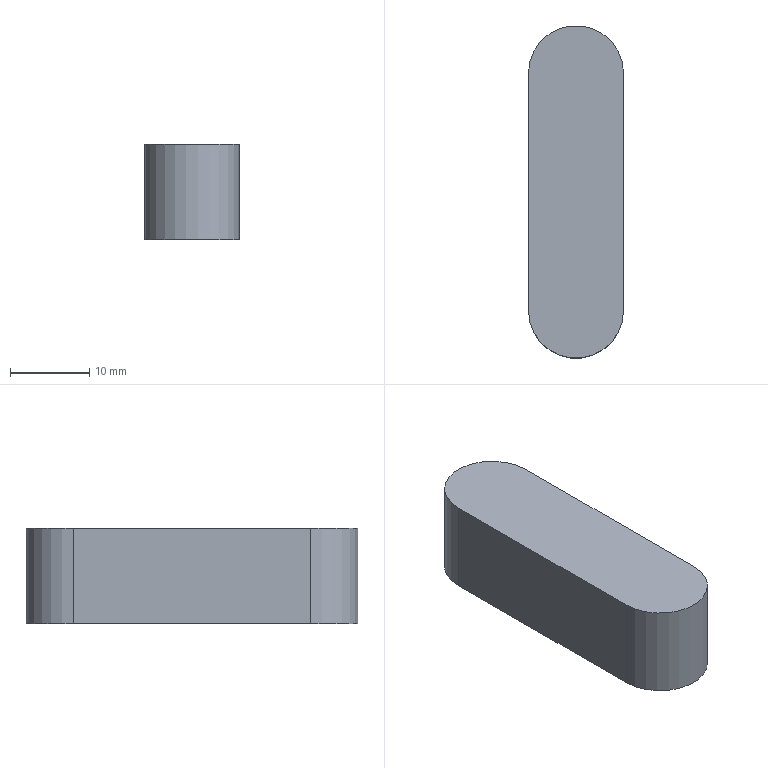Component | NX | KEY1 | 1 solid | 6 faces | box 12 x 42 x 12 mm | volume 5677 mm3 | plane 4 | cylinder 2 | commonest cylinder face diameters 12 x2
STEP:
#1=CARTESIAN_POINT('',(0.,0.,0.));
#2=DIRECTION('',(0.,0.,1.));
#3=DIRECTION('',(1.,0.,0.));
#4=AXIS2_PLACEMENT_3D('',#1,#2,#3);
#5=CARTESIAN_POINT('',(-122.42,193.257,48.472));
#6=VERTEX_POINT('',#5);
#7=CARTESIAN_POINT('',(-122.42,163.257,48.472));
#8=VERTEX_POINT('',#7);
#9=CARTESIAN_POINT('',(-122.42,178.257,48.472));
#10=DIRECTION('',(0.,-1.,0.));
#11=VECTOR('',#10,1.);
#12=LINE('',#9,#11);
#13=CARTESIAN_POINT('',(-128.42,178.257,48.472));
#14=DIRECTION('',(0.,0.,1.));
#15=DIRECTION('',(0.,-1.,0.));
#16=AXIS2_PLACEMENT_3D('',#13,#14,#15);
#17=PLANE('',#16);
#18=CARTESIAN_POINT('',(0.,6.));
#19=DIRECTION('',(1.,0.));
#20=VECTOR('',#19,1.);
#21=LINE('',#18,#20);
#22=(GEOMETRIC_REPRESENTATION_CONTEXT(2)PARAMETRIC_REPRESENTATION_CONTEXT()REPRESENTATION_CONTEXT('',''));
#23=DEFINITIONAL_REPRESENTATION('',(#21),#22);
#24=PCURVE('',#17,#23);
#25=CARTESIAN_POINT('',(-122.42,178.257,36.472));
#26=DIRECTION('',(1.,0.,0.));
#27=DIRECTION('',(0.,0.,1.));
#28=AXIS2_PLACEMENT_3D('',#25,#26,#27);
#29=PLANE('',#28);
#30=CARTESIAN_POINT('',(12.,0.));
#31=DIRECTION('',(0.,1.));
#32=VECTOR('',#31,1.);
#33=LINE('',#30,#32);
#34=(GEOMETRIC_REPRESENTATION_CONTEXT(2)PARAMETRIC_REPRESENTATION_CONTEXT()REPRESENTATION_CONTEXT('',''));
#35=DEFINITIONAL_REPRESENTATION('',(#33),#34);
#36=PCURVE('',#29,#35);
#37=SURFACE_CURVE('',#12,(#24,#36),.PCURVE_S1.);
#38=EDGE_CURVE('',#6,#8,#37,.T.);
#39=ORIENTED_EDGE('',*,*,#38,.F.);
#40=CARTESIAN_POINT('',(-134.42,193.257,48.472));
#41=VERTEX_POINT('',#40);
#42=CARTESIAN_POINT('',(-128.42,193.257,48.472));
#43=DIRECTION('',(0.,0.,1.));
#44=DIRECTION('',(0.,-1.,0.));
#45=AXIS2_PLACEMENT_3D('',#42,#43,#44);
#46=CIRCLE('',#45,6.);
#47=CARTESIAN_POINT('',(-15.,0.));
#48=DIRECTION('',(1.,0.));
#49=AXIS2_PLACEMENT_2D('',#47,#48);
#50=CIRCLE('',#49,6.);
#51=(GEOMETRIC_REPRESENTATION_CONTEXT(2)PARAMETRIC_REPRESENTATION_CONTEXT()REPRESENTATION_CONTEXT('',''));
#52=DEFINITIONAL_REPRESENTATION('',(#50),#51);
#53=PCURVE('',#17,#52);
#54=CARTESIAN_POINT('',(-128.42,193.257,36.472));
#55=DIRECTION('',(0.,0.,1.));
#56=DIRECTION('',(0.,-1.,0.));
#57=AXIS2_PLACEMENT_3D('',#54,#55,#56);
#58=CYLINDRICAL_SURFACE('',#57,6.);
#59=CARTESIAN_POINT('',(0.,12.));
#60=DIRECTION('',(1.,0.));
#61=VECTOR('',#60,1.);
#62=LINE('',#59,#61);
#63=(GEOMETRIC_REPRESENTATION_CONTEXT(2)PARAMETRIC_REPRESENTATION_CONTEXT()REPRESENTATION_CONTEXT('',''));
#64=DEFINITIONAL_REPRESENTATION('',(#62),#63);
#65=PCURVE('',#58,#64);
#66=SURFACE_CURVE('',#46,(#53,#65),.PCURVE_S1.);
#67=EDGE_CURVE('',#6,#41,#66,.T.);
#68=ORIENTED_EDGE('',*,*,#67,.T.);
#69=CARTESIAN_POINT('',(-134.42,163.257,48.472));
#70=VERTEX_POINT('',#69);
#71=CARTESIAN_POINT('',(-134.42,178.257,48.472));
#72=DIRECTION('',(0.,1.,0.));
#73=VECTOR('',#72,1.);
#74=LINE('',#71,#73);
#75=CARTESIAN_POINT('',(0.,-6.));
#76=DIRECTION('',(-1.,0.));
#77=VECTOR('',#76,1.);
#78=LINE('',#75,#77);
#79=(GEOMETRIC_REPRESENTATION_CONTEXT(2)PARAMETRIC_REPRESENTATION_CONTEXT()REPRESENTATION_CONTEXT('',''));
#80=DEFINITIONAL_REPRESENTATION('',(#78),#79);
#81=PCURVE('',#17,#80);
#82=CARTESIAN_POINT('',(-134.42,178.257,36.472));
#83=DIRECTION('',(-1.,0.,0.));
#84=DIRECTION('',(0.,0.,-1.));
#85=AXIS2_PLACEMENT_3D('',#82,#83,#84);
#86=PLANE('',#85);
#87=CARTESIAN_POINT('',(-12.,0.));
#88=DIRECTION('',(0.,-1.));
#89=VECTOR('',#88,1.);
#90=LINE('',#87,#89);
#91=(GEOMETRIC_REPRESENTATION_CONTEXT(2)PARAMETRIC_REPRESENTATION_CONTEXT()REPRESENTATION_CONTEXT('',''));
#92=DEFINITIONAL_REPRESENTATION('',(#90),#91);
#93=PCURVE('',#86,#92);
#94=SURFACE_CURVE('',#74,(#81,#93),.PCURVE_S1.);
#95=EDGE_CURVE('',#70,#41,#94,.T.);
#96=ORIENTED_EDGE('',*,*,#95,.F.);
#97=CARTESIAN_POINT('',(-128.42,163.257,48.472));
#98=DIRECTION('',(0.,0.,1.));
#99=DIRECTION('',(0.,-1.,0.));
#100=AXIS2_PLACEMENT_3D('',#97,#98,#99);
#101=CIRCLE('',#100,6.);
#102=CARTESIAN_POINT('',(15.,0.));
#103=DIRECTION('',(1.,0.));
#104=AXIS2_PLACEMENT_2D('',#102,#103);
#105=CIRCLE('',#104,6.);
#106=(GEOMETRIC_REPRESENTATION_CONTEXT(2)PARAMETRIC_REPRESENTATION_CONTEXT()REPRESENTATION_CONTEXT('',''));
#107=DEFINITIONAL_REPRESENTATION('',(#105),#106);
#108=PCURVE('',#17,#107);
#109=CARTESIAN_POINT('',(-128.42,163.257,36.472));
#110=DIRECTION('',(0.,0.,1.));
#111=DIRECTION('',(0.,-1.,0.));
#112=AXIS2_PLACEMENT_3D('',#109,#110,#111);
#113=CYLINDRICAL_SURFACE('',#112,6.);
#114=CARTESIAN_POINT('',(0.,12.));
#115=DIRECTION('',(1.,0.));
#116=VECTOR('',#115,1.);
#117=LINE('',#114,#116);
#118=(GEOMETRIC_REPRESENTATION_CONTEXT(2)PARAMETRIC_REPRESENTATION_CONTEXT()REPRESENTATION_CONTEXT('',''));
#119=DEFINITIONAL_REPRESENTATION('',(#117),#118);
#120=PCURVE('',#113,#119);
#121=SURFACE_CURVE('',#101,(#108,#120),.PCURVE_S1.);
#122=EDGE_CURVE('',#70,#8,#121,.T.);
#123=ORIENTED_EDGE('',*,*,#122,.T.);
#124=EDGE_LOOP('',(#39,#68,#96,#123));
#125=FACE_BOUND('',#124,.T.);
#126=ADVANCED_FACE('',(#125),#17,.T.);
#127=ORIENTED_EDGE('',*,*,#95,.T.);
#128=CARTESIAN_POINT('',(-134.42,193.257,36.472));
#129=VERTEX_POINT('',#128);
#130=CARTESIAN_POINT('',(-134.42,193.257,36.472));
#131=DIRECTION('',(0.,0.,-1.));
#132=VECTOR('',#131,1.);
#133=LINE('',#130,#132);
#134=CARTESIAN_POINT('',(0.,-15.));
#135=DIRECTION('',(1.,0.));
#136=VECTOR('',#135,1.);
#137=LINE('',#134,#136);
#138=(GEOMETRIC_REPRESENTATION_CONTEXT(2)PARAMETRIC_REPRESENTATION_CONTEXT()REPRESENTATION_CONTEXT('',''));
#139=DEFINITIONAL_REPRESENTATION('',(#137),#138);
#140=PCURVE('',#86,#139);
#141=CARTESIAN_POINT('',(4.712,0.));
#142=DIRECTION('',(0.,-1.));
#143=VECTOR('',#142,1.);
#144=LINE('',#141,#143);
#145=(GEOMETRIC_REPRESENTATION_CONTEXT(2)PARAMETRIC_REPRESENTATION_CONTEXT()REPRESENTATION_CONTEXT('',''));
#146=DEFINITIONAL_REPRESENTATION('',(#144),#145);
#147=PCURVE('',#58,#146);
#148=SURFACE_CURVE('',#133,(#140,#147),.PCURVE_S1.);
#149=EDGE_CURVE('',#41,#129,#148,.T.);
#150=ORIENTED_EDGE('',*,*,#149,.T.);
#151=CARTESIAN_POINT('',(-134.42,163.257,36.472));
#152=VERTEX_POINT('',#151);
#153=CARTESIAN_POINT('',(-134.42,178.257,36.472));
#154=DIRECTION('',(0.,-1.,0.));
#155=VECTOR('',#154,1.);
#156=LINE('',#153,#155);
#157=CARTESIAN_POINT('',(0.,0.));
#158=DIRECTION('',(0.,1.));
#159=VECTOR('',#158,1.);
#160=LINE('',#157,#159);
#161=(GEOMETRIC_REPRESENTATION_CONTEXT(2)PARAMETRIC_REPRESENTATION_CONTEXT()REPRESENTATION_CONTEXT('',''));
#162=DEFINITIONAL_REPRESENTATION('',(#160),#161);
#163=PCURVE('',#86,#162);
#164=CARTESIAN_POINT('',(-128.42,178.257,36.472));
#165=DIRECTION('',(0.,0.,-1.));
#166=DIRECTION('',(0.,1.,0.));
#167=AXIS2_PLACEMENT_3D('',#164,#165,#166);
#168=PLANE('',#167);
#169=CARTESIAN_POINT('',(0.,-6.));
#170=DIRECTION('',(-1.,0.));
#171=VECTOR('',#170,1.);
#172=LINE('',#169,#171);
#173=(GEOMETRIC_REPRESENTATION_CONTEXT(2)PARAMETRIC_REPRESENTATION_CONTEXT()REPRESENTATION_CONTEXT('',''));
#174=DEFINITIONAL_REPRESENTATION('',(#172),#173);
#175=PCURVE('',#168,#174);
#176=SURFACE_CURVE('',#156,(#163,#175),.PCURVE_S1.);
#177=EDGE_CURVE('',#129,#152,#176,.T.);
#178=ORIENTED_EDGE('',*,*,#177,.T.);
#179=CARTESIAN_POINT('',(-134.42,163.257,36.472));
#180=DIRECTION('',(0.,0.,1.));
#181=VECTOR('',#180,1.);
#182=LINE('',#179,#181);
#183=CARTESIAN_POINT('',(0.,15.));
#184=DIRECTION('',(-1.,0.));
#185=VECTOR('',#184,1.);
#186=LINE('',#183,#185);
#187=(GEOMETRIC_REPRESENTATION_CONTEXT(2)PARAMETRIC_REPRESENTATION_CONTEXT()REPRESENTATION_CONTEXT('',''));
#188=DEFINITIONAL_REPRESENTATION('',(#186),#187);
#189=PCURVE('',#86,#188);
#190=CARTESIAN_POINT('',(4.712,0.));
#191=DIRECTION('',(0.,1.));
#192=VECTOR('',#191,1.);
#193=LINE('',#190,#192);
#194=(GEOMETRIC_REPRESENTATION_CONTEXT(2)PARAMETRIC_REPRESENTATION_CONTEXT()REPRESENTATION_CONTEXT('',''));
#195=DEFINITIONAL_REPRESENTATION('',(#193),#194);
#196=PCURVE('',#113,#195);
#197=SURFACE_CURVE('',#182,(#189,#196),.PCURVE_S1.);
#198=EDGE_CURVE('',#152,#70,#197,.T.);
#199=ORIENTED_EDGE('',*,*,#198,.T.);
#200=EDGE_LOOP('',(#127,#150,#178,#199));
#201=FACE_BOUND('',#200,.T.);
#202=ADVANCED_FACE('',(#201),#86,.T.);
#203=CARTESIAN_POINT('',(-122.42,163.257,36.472));
#204=VERTEX_POINT('',#203);
#205=CARTESIAN_POINT('',(-122.42,193.257,36.472));
#206=VERTEX_POINT('',#205);
#207=CARTESIAN_POINT('',(-122.42,178.257,36.472));
#208=DIRECTION('',(0.,1.,0.));
#209=VECTOR('',#208,1.);
#210=LINE('',#207,#209);
#211=CARTESIAN_POINT('',(0.,0.));
#212=DIRECTION('',(0.,-1.));
#213=VECTOR('',#212,1.);
#214=LINE('',#211,#213);
#215=(GEOMETRIC_REPRESENTATION_CONTEXT(2)PARAMETRIC_REPRESENTATION_CONTEXT()REPRESENTATION_CONTEXT('',''));
#216=DEFINITIONAL_REPRESENTATION('',(#214),#215);
#217=PCURVE('',#29,#216);
#218=CARTESIAN_POINT('',(0.,6.));
#219=DIRECTION('',(1.,0.));
#220=VECTOR('',#219,1.);
#221=LINE('',#218,#220);
#222=(GEOMETRIC_REPRESENTATION_CONTEXT(2)PARAMETRIC_REPRESENTATION_CONTEXT()REPRESENTATION_CONTEXT('',''));
#223=DEFINITIONAL_REPRESENTATION('',(#221),#222);
#224=PCURVE('',#168,#223);
#225=SURFACE_CURVE('',#210,(#217,#224),.PCURVE_S1.);
#226=EDGE_CURVE('',#204,#206,#225,.T.);
#227=ORIENTED_EDGE('',*,*,#226,.T.);
#228=CARTESIAN_POINT('',(-122.42,193.257,36.472));
#229=DIRECTION('',(0.,0.,1.));
#230=VECTOR('',#229,1.);
#231=LINE('',#228,#230);
#232=CARTESIAN_POINT('',(0.,-15.));
#233=DIRECTION('',(1.,0.));
#234=VECTOR('',#233,1.);
#235=LINE('',#232,#234);
#236=(GEOMETRIC_REPRESENTATION_CONTEXT(2)PARAMETRIC_REPRESENTATION_CONTEXT()REPRESENTATION_CONTEXT('',''));
#237=DEFINITIONAL_REPRESENTATION('',(#235),#236);
#238=PCURVE('',#29,#237);
#239=CARTESIAN_POINT('',(1.571,0.));
#240=DIRECTION('',(0.,1.));
#241=VECTOR('',#240,1.);
#242=LINE('',#239,#241);
#243=(GEOMETRIC_REPRESENTATION_CONTEXT(2)PARAMETRIC_REPRESENTATION_CONTEXT()REPRESENTATION_CONTEXT('',''));
#244=DEFINITIONAL_REPRESENTATION('',(#242),#243);
#245=PCURVE('',#58,#244);
#246=SURFACE_CURVE('',#231,(#238,#245),.PCURVE_S1.);
#247=EDGE_CURVE('',#206,#6,#246,.T.);
#248=ORIENTED_EDGE('',*,*,#247,.T.);
#249=ORIENTED_EDGE('',*,*,#38,.T.);
#250=CARTESIAN_POINT('',(-122.42,163.257,36.472));
#251=DIRECTION('',(0.,0.,-1.));
#252=VECTOR('',#251,1.);
#253=LINE('',#250,#252);
#254=CARTESIAN_POINT('',(0.,15.));
#255=DIRECTION('',(-1.,0.));
#256=VECTOR('',#255,1.);
#257=LINE('',#254,#256);
#258=(GEOMETRIC_REPRESENTATION_CONTEXT(2)PARAMETRIC_REPRESENTATION_CONTEXT()REPRESENTATION_CONTEXT('',''));
#259=DEFINITIONAL_REPRESENTATION('',(#257),#258);
#260=PCURVE('',#29,#259);
#261=CARTESIAN_POINT('',(7.854,0.));
#262=DIRECTION('',(0.,-1.));
#263=VECTOR('',#262,1.);
#264=LINE('',#261,#263);
#265=(GEOMETRIC_REPRESENTATION_CONTEXT(2)PARAMETRIC_REPRESENTATION_CONTEXT()REPRESENTATION_CONTEXT('',''));
#266=DEFINITIONAL_REPRESENTATION('',(#264),#265);
#267=PCURVE('',#113,#266);
#268=SURFACE_CURVE('',#253,(#260,#267),.PCURVE_S1.);
#269=EDGE_CURVE('',#8,#204,#268,.T.);
#270=ORIENTED_EDGE('',*,*,#269,.T.);
#271=EDGE_LOOP('',(#227,#248,#249,#270));
#272=FACE_BOUND('',#271,.T.);
#273=ADVANCED_FACE('',(#272),#29,.T.);
#274=CARTESIAN_POINT('',(-128.42,193.257,36.472));
#275=DIRECTION('',(0.,0.,-1.));
#276=DIRECTION('',(0.,1.,0.));
#277=AXIS2_PLACEMENT_3D('',#274,#275,#276);
#278=CIRCLE('',#277,6.);
#279=CARTESIAN_POINT('',(15.,0.));
#280=DIRECTION('',(1.,0.));
#281=AXIS2_PLACEMENT_2D('',#279,#280);
#282=CIRCLE('',#281,6.);
#283=(GEOMETRIC_REPRESENTATION_CONTEXT(2)PARAMETRIC_REPRESENTATION_CONTEXT()REPRESENTATION_CONTEXT('',''));
#284=DEFINITIONAL_REPRESENTATION('',(#282),#283);
#285=PCURVE('',#168,#284);
#286=CARTESIAN_POINT('',(9.425,0.));
#287=DIRECTION('',(-1.,0.));
#288=VECTOR('',#287,1.);
#289=LINE('',#286,#288);
#290=(GEOMETRIC_REPRESENTATION_CONTEXT(2)PARAMETRIC_REPRESENTATION_CONTEXT()REPRESENTATION_CONTEXT('',''));
#291=DEFINITIONAL_REPRESENTATION('',(#289),#290);
#292=PCURVE('',#58,#291);
#293=SURFACE_CURVE('',#278,(#285,#292),.PCURVE_S1.);
#294=EDGE_CURVE('',#129,#206,#293,.T.);
#295=ORIENTED_EDGE('',*,*,#294,.T.);
#296=ORIENTED_EDGE('',*,*,#226,.F.);
#297=CARTESIAN_POINT('',(-128.42,163.257,36.472));
#298=DIRECTION('',(0.,0.,-1.));
#299=DIRECTION('',(0.,1.,0.));
#300=AXIS2_PLACEMENT_3D('',#297,#298,#299);
#301=CIRCLE('',#300,6.);
#302=CARTESIAN_POINT('',(-15.,0.));
#303=DIRECTION('',(1.,0.));
#304=AXIS2_PLACEMENT_2D('',#302,#303);
#305=CIRCLE('',#304,6.);
#306=(GEOMETRIC_REPRESENTATION_CONTEXT(2)PARAMETRIC_REPRESENTATION_CONTEXT()REPRESENTATION_CONTEXT('',''));
#307=DEFINITIONAL_REPRESENTATION('',(#305),#306);
#308=PCURVE('',#168,#307);
#309=CARTESIAN_POINT('',(9.425,0.));
#310=DIRECTION('',(-1.,0.));
#311=VECTOR('',#310,1.);
#312=LINE('',#309,#311);
#313=(GEOMETRIC_REPRESENTATION_CONTEXT(2)PARAMETRIC_REPRESENTATION_CONTEXT()REPRESENTATION_CONTEXT('',''));
#314=DEFINITIONAL_REPRESENTATION('',(#312),#313);
#315=PCURVE('',#113,#314);
#316=SURFACE_CURVE('',#301,(#308,#315),.PCURVE_S1.);
#317=EDGE_CURVE('',#204,#152,#316,.T.);
#318=ORIENTED_EDGE('',*,*,#317,.T.);
#319=ORIENTED_EDGE('',*,*,#177,.F.);
#320=EDGE_LOOP('',(#295,#296,#318,#319));
#321=FACE_BOUND('',#320,.T.);
#322=ADVANCED_FACE('',(#321),#168,.T.);
#323=ORIENTED_EDGE('',*,*,#67,.F.);
#324=ORIENTED_EDGE('',*,*,#247,.F.);
#325=ORIENTED_EDGE('',*,*,#294,.F.);
#326=ORIENTED_EDGE('',*,*,#149,.F.);
#327=EDGE_LOOP('',(#323,#324,#325,#326));
#328=FACE_BOUND('',#327,.T.);
#329=ADVANCED_FACE('',(#328),#58,.T.);
#330=ORIENTED_EDGE('',*,*,#122,.F.);
#331=ORIENTED_EDGE('',*,*,#198,.F.);
#332=ORIENTED_EDGE('',*,*,#317,.F.);
#333=ORIENTED_EDGE('',*,*,#269,.F.);
#334=EDGE_LOOP('',(#330,#331,#332,#333));
#335=FACE_BOUND('',#334,.T.);
#336=ADVANCED_FACE('',(#335),#113,.T.);
#337=CLOSED_SHELL('',(#126,#202,#273,#322,#329,#336));
#338=MANIFOLD_SOLID_BREP('',#337);
#339=(LENGTH_UNIT()NAMED_UNIT(*)SI_UNIT(.MILLI.,.METRE.));
#340=UNCERTAINTY_MEASURE_WITH_UNIT(LENGTH_MEASURE(0.0000001),#339,'','');
#341=(NAMED_UNIT(*)PLANE_ANGLE_UNIT()SI_UNIT($,.RADIAN.));
#342=(NAMED_UNIT(*)SI_UNIT($,.STERADIAN.)SOLID_ANGLE_UNIT());
#343=(GEOMETRIC_REPRESENTATION_CONTEXT(3)GLOBAL_UNCERTAINTY_ASSIGNED_CONTEXT((#340))GLOBAL_UNIT_ASSIGNED_CONTEXT((#339,#341,#342))REPRESENTATION_CONTEXT('',''));
#344=ADVANCED_BREP_SHAPE_REPRESENTATION('',(#4,#338),#343);